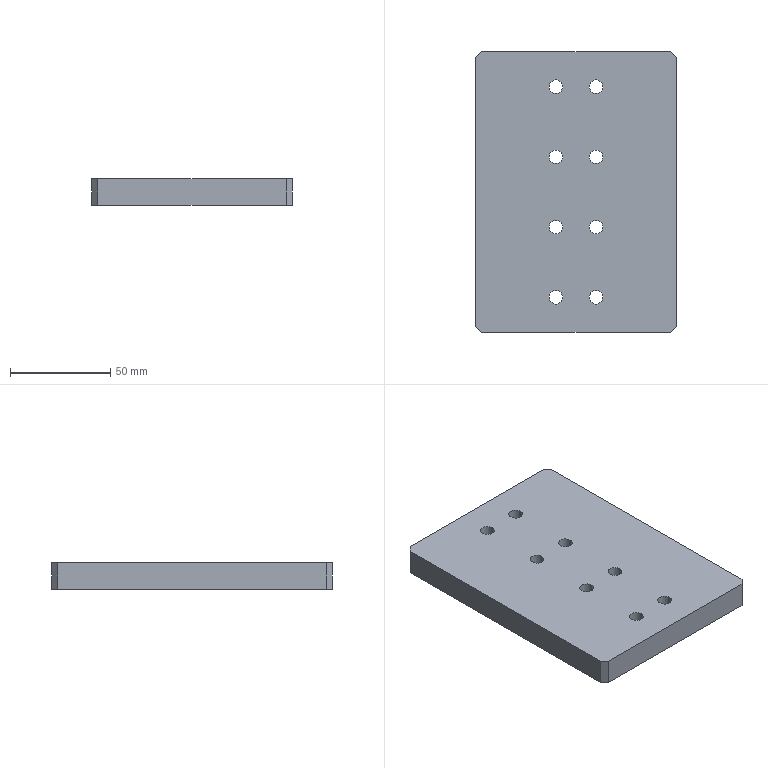Component | SolidWorks | STE21014.01-43-1 | 1 solid | 26 faces | box 100 x 140 x 13 mm | volume 177989 mm3 | cylinder 16 | plane 10 | commonest cylinder face diameters 6.8 x16 | material Q235
build123d program:
from build123d import *

# Parameters (mm, degrees)
SKETCH1_W           = 140
SKETCH1_H           = 100
BOSS_EXTRUDE1_DEPTH = 13
M8_TAPPED_HOLE1_D   = 6.8
CHAMFER1_SIZE       = 3


with BuildPart() as part:
    # Sketch1 → Boss-Extrude1 (new body)
    with BuildSketch(Plane(origin=(0, 0, 0), x_dir=(1, 0, 0), z_dir=(0, 1, 0))):
        Rectangle(SKETCH1_W, SKETCH1_H)
    extrude(amount=BOSS_EXTRUDE1_DEPTH)

    # M8 Tapped Hole1 (through all)
    with Locations(Plane(origin=(0, 13, 0), x_dir=(1, 0, 0), z_dir=(0, 1, 0))):
        with Locations((-52.5, -10), (-17.5, -10), (17.5, -10), (52.5, -10), (52.5, 10), (17.5, 10), (-17.5, 10), (-52.5, 10)):
            Hole(M8_TAPPED_HOLE1_D / 2)

    # Chamfer1
    chamfer1_edges = [part.edges().sort_by_distance(p)[0] for p in [
        (-70, 6.5, -50),
        (70, 6.5, -50),
        (70, 6.5, 50),
        (-70, 6.5, 50),
    ]]
    chamfer(chamfer1_edges, length=CHAMFER1_SIZE)


solid = part.part

# Placed as in the assembly
solid = solid.moved(Location((355, 550, -623), (90, -90, 0)))
STEP:
#1=COLOUR_RGB('',0.7922,0.8196,0.9333);
#2=FILL_AREA_STYLE_COLOUR('',#1);
#3=FILL_AREA_STYLE('',(#2));
#4=SURFACE_STYLE_FILL_AREA(#3);
#5=SURFACE_SIDE_STYLE('',(#4));
#6=SURFACE_STYLE_USAGE(.BOTH.,#5);
#7=PRESENTATION_STYLE_ASSIGNMENT((#6));
#8=CARTESIAN_POINT('',(13.717,19.587,-24.016));
#9=VERTEX_POINT('',#8);
#10=CARTESIAN_POINT('',(13.449,19.587,-24.016));
#11=VERTEX_POINT('',#10);
#12=CARTESIAN_POINT('',(13.583,19.587,-24.016));
#13=DIRECTION('',(0.,-0.,-1.));
#14=DIRECTION('',(-1.,0.,0.));
#15=AXIS2_PLACEMENT_3D('',#12,#13,#14);
#16=CIRCLE('',#15,0.1339);
#17=EDGE_CURVE('',#9,#11,#16,.T.);
#18=ORIENTED_EDGE('',*,*,#17,.F.);
#19=CARTESIAN_POINT('',(13.717,19.587,-24.528));
#20=VERTEX_POINT('',#19);
#21=CARTESIAN_POINT('',(13.717,19.587,-24.528));
#22=DIRECTION('',(0.,-0.,-1.));
#23=VECTOR('',#22,39.37);
#24=LINE('',#21,#23);
#25=EDGE_CURVE('',#9,#20,#24,.T.);
#26=ORIENTED_EDGE('',*,*,#25,.T.);
#27=CARTESIAN_POINT('',(13.449,19.587,-24.528));
#28=VERTEX_POINT('',#27);
#29=CARTESIAN_POINT('',(13.583,19.587,-24.528));
#30=DIRECTION('',(0.,-0.,-1.));
#31=DIRECTION('',(-1.,0.,0.));
#32=AXIS2_PLACEMENT_3D('',#29,#30,#31);
#33=CIRCLE('',#32,0.1339);
#34=EDGE_CURVE('',#20,#28,#33,.T.);
#35=ORIENTED_EDGE('',*,*,#34,.T.);
#36=CARTESIAN_POINT('',(13.449,19.587,-24.528));
#37=DIRECTION('',(0.,-0.,-1.));
#38=VECTOR('',#37,39.37);
#39=LINE('',#36,#38);
#40=EDGE_CURVE('',#11,#28,#39,.T.);
#41=ORIENTED_EDGE('',*,*,#40,.F.);
#42=EDGE_LOOP('',(#18,#26,#35,#41));
#43=FACE_OUTER_BOUND('',#42,.T.);
#44=CARTESIAN_POINT('',(13.583,19.587,-24.528));
#45=DIRECTION('',(0.,-0.,-1.));
#46=DIRECTION('',(-1.,0.,0.));
#47=AXIS2_PLACEMENT_3D('',#44,#45,#46);
#48=CYLINDRICAL_SURFACE('',#47,0.1339);
#49=ADVANCED_FACE('',(#43),#48,.F.);
#50=CARTESIAN_POINT('',(13.717,20.965,-24.016));
#51=VERTEX_POINT('',#50);
#52=CARTESIAN_POINT('',(13.449,20.965,-24.016));
#53=VERTEX_POINT('',#52);
#54=CARTESIAN_POINT('',(13.583,20.965,-24.016));
#55=DIRECTION('',(0.,-0.,-1.));
#56=DIRECTION('',(-1.,0.,0.));
#57=AXIS2_PLACEMENT_3D('',#54,#55,#56);
#58=CIRCLE('',#57,0.1339);
#59=EDGE_CURVE('',#51,#53,#58,.T.);
#60=ORIENTED_EDGE('',*,*,#59,.F.);
#61=CARTESIAN_POINT('',(13.717,20.965,-24.528));
#62=VERTEX_POINT('',#61);
#63=CARTESIAN_POINT('',(13.717,20.965,-24.528));
#64=DIRECTION('',(0.,-0.,-1.));
#65=VECTOR('',#64,39.37);
#66=LINE('',#63,#65);
#67=EDGE_CURVE('',#51,#62,#66,.T.);
#68=ORIENTED_EDGE('',*,*,#67,.T.);
#69=CARTESIAN_POINT('',(13.449,20.965,-24.528));
#70=VERTEX_POINT('',#69);
#71=CARTESIAN_POINT('',(13.583,20.965,-24.528));
#72=DIRECTION('',(0.,-0.,-1.));
#73=DIRECTION('',(-1.,0.,0.));
#74=AXIS2_PLACEMENT_3D('',#71,#72,#73);
#75=CIRCLE('',#74,0.1339);
#76=EDGE_CURVE('',#62,#70,#75,.T.);
#77=ORIENTED_EDGE('',*,*,#76,.T.);
#78=CARTESIAN_POINT('',(13.449,20.965,-24.528));
#79=DIRECTION('',(0.,-0.,-1.));
#80=VECTOR('',#79,39.37);
#81=LINE('',#78,#80);
#82=EDGE_CURVE('',#53,#70,#81,.T.);
#83=ORIENTED_EDGE('',*,*,#82,.F.);
#84=EDGE_LOOP('',(#60,#68,#77,#83));
#85=FACE_OUTER_BOUND('',#84,.T.);
#86=CARTESIAN_POINT('',(13.583,20.965,-24.528));
#87=DIRECTION('',(0.,-0.,-1.));
#88=DIRECTION('',(-1.,0.,0.));
#89=AXIS2_PLACEMENT_3D('',#86,#87,#88);
#90=CYLINDRICAL_SURFACE('',#89,0.1339);
#91=ADVANCED_FACE('',(#85),#90,.F.);
#92=CARTESIAN_POINT('',(13.717,22.343,-24.016));
#93=VERTEX_POINT('',#92);
#94=CARTESIAN_POINT('',(13.449,22.343,-24.016));
#95=VERTEX_POINT('',#94);
#96=CARTESIAN_POINT('',(13.583,22.343,-24.016));
#97=DIRECTION('',(0.,-0.,-1.));
#98=DIRECTION('',(-1.,0.,0.));
#99=AXIS2_PLACEMENT_3D('',#96,#97,#98);
#100=CIRCLE('',#99,0.1339);
#101=EDGE_CURVE('',#93,#95,#100,.T.);
#102=ORIENTED_EDGE('',*,*,#101,.F.);
#103=CARTESIAN_POINT('',(13.717,22.343,-24.528));
#104=VERTEX_POINT('',#103);
#105=CARTESIAN_POINT('',(13.717,22.343,-24.528));
#106=DIRECTION('',(0.,-0.,-1.));
#107=VECTOR('',#106,39.37);
#108=LINE('',#105,#107);
#109=EDGE_CURVE('',#93,#104,#108,.T.);
#110=ORIENTED_EDGE('',*,*,#109,.T.);
#111=CARTESIAN_POINT('',(13.449,22.343,-24.528));
#112=VERTEX_POINT('',#111);
#113=CARTESIAN_POINT('',(13.583,22.343,-24.528));
#114=DIRECTION('',(0.,-0.,-1.));
#115=DIRECTION('',(-1.,0.,0.));
#116=AXIS2_PLACEMENT_3D('',#113,#114,#115);
#117=CIRCLE('',#116,0.1339);
#118=EDGE_CURVE('',#104,#112,#117,.T.);
#119=ORIENTED_EDGE('',*,*,#118,.T.);
#120=CARTESIAN_POINT('',(13.449,22.343,-24.528));
#121=DIRECTION('',(0.,-0.,-1.));
#122=VECTOR('',#121,39.37);
#123=LINE('',#120,#122);
#124=EDGE_CURVE('',#95,#112,#123,.T.);
#125=ORIENTED_EDGE('',*,*,#124,.F.);
#126=EDGE_LOOP('',(#102,#110,#119,#125));
#127=FACE_OUTER_BOUND('',#126,.T.);
#128=CARTESIAN_POINT('',(13.583,22.343,-24.528));
#129=DIRECTION('',(0.,-0.,-1.));
#130=DIRECTION('',(-1.,0.,0.));
#131=AXIS2_PLACEMENT_3D('',#128,#129,#130);
#132=CYLINDRICAL_SURFACE('',#131,0.1339);
#133=ADVANCED_FACE('',(#127),#132,.F.);
#134=CARTESIAN_POINT('',(13.717,23.72,-24.016));
#135=VERTEX_POINT('',#134);
#136=CARTESIAN_POINT('',(13.449,23.72,-24.016));
#137=VERTEX_POINT('',#136);
#138=CARTESIAN_POINT('',(13.583,23.72,-24.016));
#139=DIRECTION('',(0.,-0.,-1.));
#140=DIRECTION('',(-1.,0.,0.));
#141=AXIS2_PLACEMENT_3D('',#138,#139,#140);
#142=CIRCLE('',#141,0.1339);
#143=EDGE_CURVE('',#135,#137,#142,.T.);
#144=ORIENTED_EDGE('',*,*,#143,.F.);
#145=CARTESIAN_POINT('',(13.717,23.72,-24.528));
#146=VERTEX_POINT('',#145);
#147=CARTESIAN_POINT('',(13.717,23.72,-24.528));
#148=DIRECTION('',(0.,-0.,-1.));
#149=VECTOR('',#148,39.37);
#150=LINE('',#147,#149);
#151=EDGE_CURVE('',#135,#146,#150,.T.);
#152=ORIENTED_EDGE('',*,*,#151,.T.);
#153=CARTESIAN_POINT('',(13.449,23.72,-24.528));
#154=VERTEX_POINT('',#153);
#155=CARTESIAN_POINT('',(13.583,23.72,-24.528));
#156=DIRECTION('',(0.,-0.,-1.));
#157=DIRECTION('',(-1.,0.,0.));
#158=AXIS2_PLACEMENT_3D('',#155,#156,#157);
#159=CIRCLE('',#158,0.1339);
#160=EDGE_CURVE('',#146,#154,#159,.T.);
#161=ORIENTED_EDGE('',*,*,#160,.T.);
#162=CARTESIAN_POINT('',(13.449,23.72,-24.528));
#163=DIRECTION('',(0.,-0.,-1.));
#164=VECTOR('',#163,39.37);
#165=LINE('',#162,#164);
#166=EDGE_CURVE('',#137,#154,#165,.T.);
#167=ORIENTED_EDGE('',*,*,#166,.F.);
#168=EDGE_LOOP('',(#144,#152,#161,#167));
#169=FACE_OUTER_BOUND('',#168,.T.);
#170=CARTESIAN_POINT('',(13.583,23.72,-24.528));
#171=DIRECTION('',(0.,-0.,-1.));
#172=DIRECTION('',(-1.,0.,0.));
#173=AXIS2_PLACEMENT_3D('',#170,#171,#172);
#174=CYLINDRICAL_SURFACE('',#173,0.1339);
#175=ADVANCED_FACE('',(#169),#174,.F.);
#176=CARTESIAN_POINT('',(14.504,23.72,-24.016));
#177=VERTEX_POINT('',#176);
#178=CARTESIAN_POINT('',(14.236,23.72,-24.016));
#179=VERTEX_POINT('',#178);
#180=CARTESIAN_POINT('',(14.37,23.72,-24.016));
#181=DIRECTION('',(0.,-0.,-1.));
#182=DIRECTION('',(-1.,0.,0.));
#183=AXIS2_PLACEMENT_3D('',#180,#181,#182);
#184=CIRCLE('',#183,0.1339);
#185=EDGE_CURVE('',#177,#179,#184,.T.);
#186=ORIENTED_EDGE('',*,*,#185,.F.);
#187=CARTESIAN_POINT('',(14.504,23.72,-24.528));
#188=VERTEX_POINT('',#187);
#189=CARTESIAN_POINT('',(14.504,23.72,-24.528));
#190=DIRECTION('',(0.,-0.,-1.));
#191=VECTOR('',#190,39.37);
#192=LINE('',#189,#191);
#193=EDGE_CURVE('',#177,#188,#192,.T.);
#194=ORIENTED_EDGE('',*,*,#193,.T.);
#195=CARTESIAN_POINT('',(14.236,23.72,-24.528));
#196=VERTEX_POINT('',#195);
#197=CARTESIAN_POINT('',(14.37,23.72,-24.528));
#198=DIRECTION('',(0.,-0.,-1.));
#199=DIRECTION('',(-1.,0.,0.));
#200=AXIS2_PLACEMENT_3D('',#197,#198,#199);
#201=CIRCLE('',#200,0.1339);
#202=EDGE_CURVE('',#188,#196,#201,.T.);
#203=ORIENTED_EDGE('',*,*,#202,.T.);
#204=CARTESIAN_POINT('',(14.236,23.72,-24.528));
#205=DIRECTION('',(0.,-0.,-1.));
#206=VECTOR('',#205,39.37);
#207=LINE('',#204,#206);
#208=EDGE_CURVE('',#179,#196,#207,.T.);
#209=ORIENTED_EDGE('',*,*,#208,.F.);
#210=EDGE_LOOP('',(#186,#194,#203,#209));
#211=FACE_OUTER_BOUND('',#210,.T.);
#212=CARTESIAN_POINT('',(14.37,23.72,-24.528));
#213=DIRECTION('',(0.,-0.,-1.));
#214=DIRECTION('',(-1.,0.,0.));
#215=AXIS2_PLACEMENT_3D('',#212,#213,#214);
#216=CYLINDRICAL_SURFACE('',#215,0.1339);
#217=ADVANCED_FACE('',(#211),#216,.F.);
#218=CARTESIAN_POINT('',(14.504,22.343,-24.016));
#219=VERTEX_POINT('',#218);
#220=CARTESIAN_POINT('',(14.236,22.343,-24.016));
#221=VERTEX_POINT('',#220);
#222=CARTESIAN_POINT('',(14.37,22.343,-24.016));
#223=DIRECTION('',(0.,-0.,-1.));
#224=DIRECTION('',(-1.,0.,0.));
#225=AXIS2_PLACEMENT_3D('',#222,#223,#224);
#226=CIRCLE('',#225,0.1339);
#227=EDGE_CURVE('',#219,#221,#226,.T.);
#228=ORIENTED_EDGE('',*,*,#227,.F.);
#229=CARTESIAN_POINT('',(14.504,22.343,-24.528));
#230=VERTEX_POINT('',#229);
#231=CARTESIAN_POINT('',(14.504,22.343,-24.528));
#232=DIRECTION('',(0.,-0.,-1.));
#233=VECTOR('',#232,39.37);
#234=LINE('',#231,#233);
#235=EDGE_CURVE('',#219,#230,#234,.T.);
#236=ORIENTED_EDGE('',*,*,#235,.T.);
#237=CARTESIAN_POINT('',(14.236,22.343,-24.528));
#238=VERTEX_POINT('',#237);
#239=CARTESIAN_POINT('',(14.37,22.343,-24.528));
#240=DIRECTION('',(0.,-0.,-1.));
#241=DIRECTION('',(-1.,0.,0.));
#242=AXIS2_PLACEMENT_3D('',#239,#240,#241);
#243=CIRCLE('',#242,0.1339);
#244=EDGE_CURVE('',#230,#238,#243,.T.);
#245=ORIENTED_EDGE('',*,*,#244,.T.);
#246=CARTESIAN_POINT('',(14.236,22.343,-24.528));
#247=DIRECTION('',(0.,-0.,-1.));
#248=VECTOR('',#247,39.37);
#249=LINE('',#246,#248);
#250=EDGE_CURVE('',#221,#238,#249,.T.);
#251=ORIENTED_EDGE('',*,*,#250,.F.);
#252=EDGE_LOOP('',(#228,#236,#245,#251));
#253=FACE_OUTER_BOUND('',#252,.T.);
#254=CARTESIAN_POINT('',(14.37,22.343,-24.528));
#255=DIRECTION('',(0.,-0.,-1.));
#256=DIRECTION('',(-1.,0.,0.));
#257=AXIS2_PLACEMENT_3D('',#254,#255,#256);
#258=CYLINDRICAL_SURFACE('',#257,0.1339);
#259=ADVANCED_FACE('',(#253),#258,.F.);
#260=CARTESIAN_POINT('',(14.504,20.965,-24.016));
#261=VERTEX_POINT('',#260);
#262=CARTESIAN_POINT('',(14.236,20.965,-24.016));
#263=VERTEX_POINT('',#262);
#264=CARTESIAN_POINT('',(14.37,20.965,-24.016));
#265=DIRECTION('',(0.,-0.,-1.));
#266=DIRECTION('',(-1.,0.,0.));
#267=AXIS2_PLACEMENT_3D('',#264,#265,#266);
#268=CIRCLE('',#267,0.1339);
#269=EDGE_CURVE('',#261,#263,#268,.T.);
#270=ORIENTED_EDGE('',*,*,#269,.F.);
#271=CARTESIAN_POINT('',(14.504,20.965,-24.528));
#272=VERTEX_POINT('',#271);
#273=CARTESIAN_POINT('',(14.504,20.965,-24.528));
#274=DIRECTION('',(0.,-0.,-1.));
#275=VECTOR('',#274,39.37);
#276=LINE('',#273,#275);
#277=EDGE_CURVE('',#261,#272,#276,.T.);
#278=ORIENTED_EDGE('',*,*,#277,.T.);
#279=CARTESIAN_POINT('',(14.236,20.965,-24.528));
#280=VERTEX_POINT('',#279);
#281=CARTESIAN_POINT('',(14.37,20.965,-24.528));
#282=DIRECTION('',(0.,-0.,-1.));
#283=DIRECTION('',(-1.,0.,0.));
#284=AXIS2_PLACEMENT_3D('',#281,#282,#283);
#285=CIRCLE('',#284,0.1339);
#286=EDGE_CURVE('',#272,#280,#285,.T.);
#287=ORIENTED_EDGE('',*,*,#286,.T.);
#288=CARTESIAN_POINT('',(14.236,20.965,-24.528));
#289=DIRECTION('',(0.,-0.,-1.));
#290=VECTOR('',#289,39.37);
#291=LINE('',#288,#290);
#292=EDGE_CURVE('',#263,#280,#291,.T.);
#293=ORIENTED_EDGE('',*,*,#292,.F.);
#294=EDGE_LOOP('',(#270,#278,#287,#293));
#295=FACE_OUTER_BOUND('',#294,.T.);
#296=CARTESIAN_POINT('',(14.37,20.965,-24.528));
#297=DIRECTION('',(0.,-0.,-1.));
#298=DIRECTION('',(-1.,0.,0.));
#299=AXIS2_PLACEMENT_3D('',#296,#297,#298);
#300=CYLINDRICAL_SURFACE('',#299,0.1339);
#301=ADVANCED_FACE('',(#295),#300,.F.);
#302=CARTESIAN_POINT('',(14.504,19.587,-24.016));
#303=VERTEX_POINT('',#302);
#304=CARTESIAN_POINT('',(14.236,19.587,-24.016));
#305=VERTEX_POINT('',#304);
#306=CARTESIAN_POINT('',(14.37,19.587,-24.016));
#307=DIRECTION('',(0.,-0.,-1.));
#308=DIRECTION('',(-1.,0.,0.));
#309=AXIS2_PLACEMENT_3D('',#306,#307,#308);
#310=CIRCLE('',#309,0.1339);
#311=EDGE_CURVE('',#303,#305,#310,.T.);
#312=ORIENTED_EDGE('',*,*,#311,.F.);
#313=CARTESIAN_POINT('',(14.504,19.587,-24.528));
#314=VERTEX_POINT('',#313);
#315=CARTESIAN_POINT('',(14.504,19.587,-24.528));
#316=DIRECTION('',(0.,-0.,-1.));
#317=VECTOR('',#316,39.37);
#318=LINE('',#315,#317);
#319=EDGE_CURVE('',#303,#314,#318,.T.);
#320=ORIENTED_EDGE('',*,*,#319,.T.);
#321=CARTESIAN_POINT('',(14.236,19.587,-24.528));
#322=VERTEX_POINT('',#321);
#323=CARTESIAN_POINT('',(14.37,19.587,-24.528));
#324=DIRECTION('',(0.,-0.,-1.));
#325=DIRECTION('',(-1.,0.,0.));
#326=AXIS2_PLACEMENT_3D('',#323,#324,#325);
#327=CIRCLE('',#326,0.1339);
#328=EDGE_CURVE('',#314,#322,#327,.T.);
#329=ORIENTED_EDGE('',*,*,#328,.T.);
#330=CARTESIAN_POINT('',(14.236,19.587,-24.528));
#331=DIRECTION('',(0.,-0.,-1.));
#332=VECTOR('',#331,39.37);
#333=LINE('',#330,#332);
#334=EDGE_CURVE('',#305,#322,#333,.T.);
#335=ORIENTED_EDGE('',*,*,#334,.F.);
#336=EDGE_LOOP('',(#312,#320,#329,#335));
#337=FACE_OUTER_BOUND('',#336,.T.);
#338=CARTESIAN_POINT('',(14.37,19.587,-24.528));
#339=DIRECTION('',(0.,-0.,-1.));
#340=DIRECTION('',(-1.,0.,0.));
#341=AXIS2_PLACEMENT_3D('',#338,#339,#340);
#342=CYLINDRICAL_SURFACE('',#341,0.1339);
#343=ADVANCED_FACE('',(#337),#342,.F.);
#344=CARTESIAN_POINT('',(15.827,18.898,-24.528));
#345=VERTEX_POINT('',#344);
#346=CARTESIAN_POINT('',(12.126,18.898,-24.528));
#347=VERTEX_POINT('',#346);
#348=CARTESIAN_POINT('',(12.008,18.898,-24.528));
#349=DIRECTION('',(-1.,0.,-0.));
#350=VECTOR('',#349,39.37);
#351=LINE('',#348,#350);
#352=EDGE_CURVE('',#345,#347,#351,.T.);
#353=ORIENTED_EDGE('',*,*,#352,.F.);
#354=CARTESIAN_POINT('',(15.827,18.898,-24.016));
#355=VERTEX_POINT('',#354);
#356=CARTESIAN_POINT('',(15.827,18.898,-24.528));
#357=DIRECTION('',(-0.,0.,1.));
#358=VECTOR('',#357,39.37);
#359=LINE('',#356,#358);
#360=EDGE_CURVE('',#345,#355,#359,.T.);
#361=ORIENTED_EDGE('',*,*,#360,.T.);
#362=CARTESIAN_POINT('',(12.126,18.898,-24.016));
#363=VERTEX_POINT('',#362);
#364=CARTESIAN_POINT('',(12.008,18.898,-24.016));
#365=DIRECTION('',(-1.,0.,-0.));
#366=VECTOR('',#365,39.37);
#367=LINE('',#364,#366);
#368=EDGE_CURVE('',#355,#363,#367,.T.);
#369=ORIENTED_EDGE('',*,*,#368,.T.);
#370=CARTESIAN_POINT('',(12.126,18.898,-24.528));
#371=DIRECTION('',(0.,-0.,-1.));
#372=VECTOR('',#371,39.37);
#373=LINE('',#370,#372);
#374=EDGE_CURVE('',#363,#347,#373,.T.);
#375=ORIENTED_EDGE('',*,*,#374,.T.);
#376=EDGE_LOOP('',(#353,#361,#369,#375));
#377=FACE_OUTER_BOUND('',#376,.T.);
#378=CARTESIAN_POINT('',(12.008,18.898,-24.528));
#379=DIRECTION('',(0.,1.,-0.));
#380=DIRECTION('',(1.,-0.,0.));
#381=AXIS2_PLACEMENT_3D('',#378,#379,#380);
#382=PLANE('',#381);
#383=ADVANCED_FACE('',(#377),#382,.F.);
#384=CARTESIAN_POINT('',(12.008,19.016,-24.016));
#385=VERTEX_POINT('',#384);
#386=CARTESIAN_POINT('',(12.008,24.291,-24.016));
#387=VERTEX_POINT('',#386);
#388=CARTESIAN_POINT('',(12.008,24.409,-24.016));
#389=DIRECTION('',(0.,1.,-0.));
#390=VECTOR('',#389,39.37);
#391=LINE('',#388,#390);
#392=EDGE_CURVE('',#385,#387,#391,.T.);
#393=ORIENTED_EDGE('',*,*,#392,.T.);
#394=CARTESIAN_POINT('',(12.008,24.291,-24.528));
#395=VERTEX_POINT('',#394);
#396=CARTESIAN_POINT('',(12.008,24.291,-24.528));
#397=DIRECTION('',(0.,-0.,-1.));
#398=VECTOR('',#397,39.37);
#399=LINE('',#396,#398);
#400=EDGE_CURVE('',#387,#395,#399,.T.);
#401=ORIENTED_EDGE('',*,*,#400,.T.);
#402=CARTESIAN_POINT('',(12.008,19.016,-24.528));
#403=VERTEX_POINT('',#402);
#404=CARTESIAN_POINT('',(12.008,24.409,-24.528));
#405=DIRECTION('',(0.,1.,-0.));
#406=VECTOR('',#405,39.37);
#407=LINE('',#404,#406);
#408=EDGE_CURVE('',#403,#395,#407,.T.);
#409=ORIENTED_EDGE('',*,*,#408,.F.);
#410=CARTESIAN_POINT('',(12.008,19.016,-24.528));
#411=DIRECTION('',(-0.,0.,1.));
#412=VECTOR('',#411,39.37);
#413=LINE('',#410,#412);
#414=EDGE_CURVE('',#403,#385,#413,.T.);
#415=ORIENTED_EDGE('',*,*,#414,.T.);
#416=EDGE_LOOP('',(#393,#401,#409,#415));
#417=FACE_OUTER_BOUND('',#416,.T.);
#418=CARTESIAN_POINT('',(12.008,24.409,-24.528));
#419=DIRECTION('',(1.,-0.,0.));
#420=DIRECTION('',(-0.,-1.,0.));
#421=AXIS2_PLACEMENT_3D('',#418,#419,#420);
#422=PLANE('',#421);
#423=ADVANCED_FACE('',(#417),#422,.F.);
#424=CARTESIAN_POINT('',(12.126,24.409,-24.528));
#425=VERTEX_POINT('',#424);
#426=CARTESIAN_POINT('',(15.827,24.409,-24.528));
#427=VERTEX_POINT('',#426);
#428=CARTESIAN_POINT('',(12.008,24.409,-24.528));
#429=DIRECTION('',(1.,-0.,0.));
#430=VECTOR('',#429,39.37);
#431=LINE('',#428,#430);
#432=EDGE_CURVE('',#425,#427,#431,.T.);
#433=ORIENTED_EDGE('',*,*,#432,.F.);
#434=CARTESIAN_POINT('',(12.126,24.409,-24.016));
#435=VERTEX_POINT('',#434);
#436=CARTESIAN_POINT('',(12.126,24.409,-24.528));
#437=DIRECTION('',(-0.,0.,1.));
#438=VECTOR('',#437,39.37);
#439=LINE('',#436,#438);
#440=EDGE_CURVE('',#425,#435,#439,.T.);
#441=ORIENTED_EDGE('',*,*,#440,.T.);
#442=CARTESIAN_POINT('',(15.827,24.409,-24.016));
#443=VERTEX_POINT('',#442);
#444=CARTESIAN_POINT('',(12.008,24.409,-24.016));
#445=DIRECTION('',(1.,-0.,0.));
#446=VECTOR('',#445,39.37);
#447=LINE('',#444,#446);
#448=EDGE_CURVE('',#435,#443,#447,.T.);
#449=ORIENTED_EDGE('',*,*,#448,.T.);
#450=CARTESIAN_POINT('',(15.827,24.409,-24.528));
#451=DIRECTION('',(0.,-0.,-1.));
#452=VECTOR('',#451,39.37);
#453=LINE('',#450,#452);
#454=EDGE_CURVE('',#443,#427,#453,.T.);
#455=ORIENTED_EDGE('',*,*,#454,.T.);
#456=EDGE_LOOP('',(#433,#441,#449,#455));
#457=FACE_OUTER_BOUND('',#456,.T.);
#458=CARTESIAN_POINT('',(12.008,24.409,-24.528));
#459=DIRECTION('',(-0.,-1.,0.));
#460=DIRECTION('',(-1.,0.,-0.));
#461=AXIS2_PLACEMENT_3D('',#458,#459,#460);
#462=PLANE('',#461);
#463=ADVANCED_FACE('',(#457),#462,.F.);
#464=CARTESIAN_POINT('',(15.945,24.291,-24.528));
#465=VERTEX_POINT('',#464);
#466=CARTESIAN_POINT('',(15.945,19.016,-24.528));
#467=VERTEX_POINT('',#466);
#468=CARTESIAN_POINT('',(15.945,24.409,-24.528));
#469=DIRECTION('',(-0.,-1.,0.));
#470=VECTOR('',#469,39.37);
#471=LINE('',#468,#470);
#472=EDGE_CURVE('',#465,#467,#471,.T.);
#473=ORIENTED_EDGE('',*,*,#472,.F.);
#474=CARTESIAN_POINT('',(15.945,24.291,-24.016));
#475=VERTEX_POINT('',#474);
#476=CARTESIAN_POINT('',(15.945,24.291,-24.528));
#477=DIRECTION('',(-0.,0.,1.));
#478=VECTOR('',#477,39.37);
#479=LINE('',#476,#478);
#480=EDGE_CURVE('',#465,#475,#479,.T.);
#481=ORIENTED_EDGE('',*,*,#480,.T.);
#482=CARTESIAN_POINT('',(15.945,19.016,-24.016));
#483=VERTEX_POINT('',#482);
#484=CARTESIAN_POINT('',(15.945,24.409,-24.016));
#485=DIRECTION('',(-0.,-1.,0.));
#486=VECTOR('',#485,39.37);
#487=LINE('',#484,#486);
#488=EDGE_CURVE('',#475,#483,#487,.T.);
#489=ORIENTED_EDGE('',*,*,#488,.T.);
#490=CARTESIAN_POINT('',(15.945,19.016,-24.528));
#491=DIRECTION('',(0.,-0.,-1.));
#492=VECTOR('',#491,39.37);
#493=LINE('',#490,#492);
#494=EDGE_CURVE('',#483,#467,#493,.T.);
#495=ORIENTED_EDGE('',*,*,#494,.T.);
#496=EDGE_LOOP('',(#473,#481,#489,#495));
#497=FACE_OUTER_BOUND('',#496,.T.);
#498=CARTESIAN_POINT('',(15.945,24.409,-24.528));
#499=DIRECTION('',(-1.,0.,-0.));
#500=DIRECTION('',(0.,1.,-0.));
#501=AXIS2_PLACEMENT_3D('',#498,#499,#500);
#502=PLANE('',#501);
#503=ADVANCED_FACE('',(#497),#502,.F.);
#504=CARTESIAN_POINT('',(13.583,19.587,-24.528));
#505=DIRECTION('',(0.,-0.,-1.));
#506=DIRECTION('',(-1.,0.,0.));
#507=AXIS2_PLACEMENT_3D('',#504,#505,#506);
#508=CIRCLE('',#507,0.1339);
#509=EDGE_CURVE('',#28,#20,#508,.T.);
#510=ORIENTED_EDGE('',*,*,#509,.F.);
#511=ORIENTED_EDGE('',*,*,#34,.F.);
#512=EDGE_LOOP('',(#510,#511));
#513=FACE_BOUND('',#512,.T.);
#514=CARTESIAN_POINT('',(13.583,20.965,-24.528));
#515=DIRECTION('',(0.,-0.,-1.));
#516=DIRECTION('',(-1.,0.,0.));
#517=AXIS2_PLACEMENT_3D('',#514,#515,#516);
#518=CIRCLE('',#517,0.1339);
#519=EDGE_CURVE('',#70,#62,#518,.T.);
#520=ORIENTED_EDGE('',*,*,#519,.F.);
#521=ORIENTED_EDGE('',*,*,#76,.F.);
#522=EDGE_LOOP('',(#520,#521));
#523=FACE_BOUND('',#522,.T.);
#524=CARTESIAN_POINT('',(13.583,22.343,-24.528));
#525=DIRECTION('',(0.,-0.,-1.));
#526=DIRECTION('',(-1.,0.,0.));
#527=AXIS2_PLACEMENT_3D('',#524,#525,#526);
#528=CIRCLE('',#527,0.1339);
#529=EDGE_CURVE('',#112,#104,#528,.T.);
#530=ORIENTED_EDGE('',*,*,#529,.F.);
#531=ORIENTED_EDGE('',*,*,#118,.F.);
#532=EDGE_LOOP('',(#530,#531));
#533=FACE_BOUND('',#532,.T.);
#534=CARTESIAN_POINT('',(13.583,23.72,-24.528));
#535=DIRECTION('',(0.,-0.,-1.));
#536=DIRECTION('',(-1.,0.,0.));
#537=AXIS2_PLACEMENT_3D('',#534,#535,#536);
#538=CIRCLE('',#537,0.1339);
#539=EDGE_CURVE('',#154,#146,#538,.T.);
#540=ORIENTED_EDGE('',*,*,#539,.F.);
#541=ORIENTED_EDGE('',*,*,#160,.F.);
#542=EDGE_LOOP('',(#540,#541));
#543=FACE_BOUND('',#542,.T.);
#544=CARTESIAN_POINT('',(14.37,23.72,-24.528));
#545=DIRECTION('',(0.,-0.,-1.));
#546=DIRECTION('',(-1.,0.,0.));
#547=AXIS2_PLACEMENT_3D('',#544,#545,#546);
#548=CIRCLE('',#547,0.1339);
#549=EDGE_CURVE('',#196,#188,#548,.T.);
#550=ORIENTED_EDGE('',*,*,#549,.F.);
#551=ORIENTED_EDGE('',*,*,#202,.F.);
#552=EDGE_LOOP('',(#550,#551));
#553=FACE_BOUND('',#552,.T.);
#554=CARTESIAN_POINT('',(14.37,22.343,-24.528));
#555=DIRECTION('',(0.,-0.,-1.));
#556=DIRECTION('',(-1.,0.,0.));
#557=AXIS2_PLACEMENT_3D('',#554,#555,#556);
#558=CIRCLE('',#557,0.1339);
#559=EDGE_CURVE('',#238,#230,#558,.T.);
#560=ORIENTED_EDGE('',*,*,#559,.F.);
#561=ORIENTED_EDGE('',*,*,#244,.F.);
#562=EDGE_LOOP('',(#560,#561));
#563=FACE_BOUND('',#562,.T.);
#564=CARTESIAN_POINT('',(14.37,20.965,-24.528));
#565=DIRECTION('',(0.,-0.,-1.));
#566=DIRECTION('',(-1.,0.,0.));
#567=AXIS2_PLACEMENT_3D('',#564,#565,#566);
#568=CIRCLE('',#567,0.1339);
#569=EDGE_CURVE('',#280,#272,#568,.T.);
#570=ORIENTED_EDGE('',*,*,#569,.F.);
#571=ORIENTED_EDGE('',*,*,#286,.F.);
#572=EDGE_LOOP('',(#570,#571));
#573=FACE_BOUND('',#572,.T.);
#574=CARTESIAN_POINT('',(14.37,19.587,-24.528));
#575=DIRECTION('',(0.,-0.,-1.));
#576=DIRECTION('',(-1.,0.,0.));
#577=AXIS2_PLACEMENT_3D('',#574,#575,#576);
#578=CIRCLE('',#577,0.1339);
#579=EDGE_CURVE('',#322,#314,#578,.T.);
#580=ORIENTED_EDGE('',*,*,#579,.F.);
#581=ORIENTED_EDGE('',*,*,#328,.F.);
#582=EDGE_LOOP('',(#580,#581));
#583=FACE_BOUND('',#582,.T.);
#584=ORIENTED_EDGE('',*,*,#408,.T.);
#585=CARTESIAN_POINT('',(11.673,23.957,-24.528));
#586=DIRECTION('',(0.7071,0.7071,-0.));
#587=VECTOR('',#586,39.37);
#588=LINE('',#585,#587);
#589=EDGE_CURVE('',#395,#425,#588,.T.);
#590=ORIENTED_EDGE('',*,*,#589,.T.);
#591=ORIENTED_EDGE('',*,*,#432,.T.);
#592=CARTESIAN_POINT('',(16.28,23.957,-24.528));
#593=DIRECTION('',(0.7071,-0.7071,0.));
#594=VECTOR('',#593,39.37);
#595=LINE('',#592,#594);
#596=EDGE_CURVE('',#427,#465,#595,.T.);
#597=ORIENTED_EDGE('',*,*,#596,.T.);
#598=ORIENTED_EDGE('',*,*,#472,.T.);
#599=CARTESIAN_POINT('',(16.28,19.35,-24.528));
#600=DIRECTION('',(-0.7071,-0.7071,0.));
#601=VECTOR('',#600,39.37);
#602=LINE('',#599,#601);
#603=EDGE_CURVE('',#467,#345,#602,.T.);
#604=ORIENTED_EDGE('',*,*,#603,.T.);
#605=ORIENTED_EDGE('',*,*,#352,.T.);
#606=CARTESIAN_POINT('',(11.673,19.35,-24.528));
#607=DIRECTION('',(-0.7071,0.7071,-0.));
#608=VECTOR('',#607,39.37);
#609=LINE('',#606,#608);
#610=EDGE_CURVE('',#347,#403,#609,.T.);
#611=ORIENTED_EDGE('',*,*,#610,.T.);
#612=EDGE_LOOP('',(#584,#590,#591,#597,#598,#604,#605,#611));
#613=FACE_OUTER_BOUND('',#612,.T.);
#614=CARTESIAN_POINT('',(13.976,21.654,-24.528));
#615=DIRECTION('',(0.,-0.,-1.));
#616=DIRECTION('',(-1.,0.,-0.));
#617=AXIS2_PLACEMENT_3D('',#614,#615,#616);
#618=PLANE('',#617);
#619=ADVANCED_FACE('',(#513,#523,#533,#543,#553,#563,#573,#583,#613),#618,.T.);
#620=CARTESIAN_POINT('',(13.583,19.587,-24.016));
#621=DIRECTION('',(0.,-0.,-1.));
#622=DIRECTION('',(-1.,0.,0.));
#623=AXIS2_PLACEMENT_3D('',#620,#621,#622);
#624=CIRCLE('',#623,0.1339);
#625=EDGE_CURVE('',#11,#9,#624,.T.);
#626=ORIENTED_EDGE('',*,*,#625,.T.);
#627=ORIENTED_EDGE('',*,*,#17,.T.);
#628=EDGE_LOOP('',(#626,#627));
#629=FACE_BOUND('',#628,.T.);
#630=CARTESIAN_POINT('',(13.583,20.965,-24.016));
#631=DIRECTION('',(0.,-0.,-1.));
#632=DIRECTION('',(-1.,0.,0.));
#633=AXIS2_PLACEMENT_3D('',#630,#631,#632);
#634=CIRCLE('',#633,0.1339);
#635=EDGE_CURVE('',#53,#51,#634,.T.);
#636=ORIENTED_EDGE('',*,*,#635,.T.);
#637=ORIENTED_EDGE('',*,*,#59,.T.);
#638=EDGE_LOOP('',(#636,#637));
#639=FACE_BOUND('',#638,.T.);
#640=CARTESIAN_POINT('',(13.583,22.343,-24.016));
#641=DIRECTION('',(0.,-0.,-1.));
#642=DIRECTION('',(-1.,0.,0.));
#643=AXIS2_PLACEMENT_3D('',#640,#641,#642);
#644=CIRCLE('',#643,0.1339);
#645=EDGE_CURVE('',#95,#93,#644,.T.);
#646=ORIENTED_EDGE('',*,*,#645,.T.);
#647=ORIENTED_EDGE('',*,*,#101,.T.);
#648=EDGE_LOOP('',(#646,#647));
#649=FACE_BOUND('',#648,.T.);
#650=CARTESIAN_POINT('',(13.583,23.72,-24.016));
#651=DIRECTION('',(0.,-0.,-1.));
#652=DIRECTION('',(-1.,0.,0.));
#653=AXIS2_PLACEMENT_3D('',#650,#651,#652);
#654=CIRCLE('',#653,0.1339);
#655=EDGE_CURVE('',#137,#135,#654,.T.);
#656=ORIENTED_EDGE('',*,*,#655,.T.);
#657=ORIENTED_EDGE('',*,*,#143,.T.);
#658=EDGE_LOOP('',(#656,#657));
#659=FACE_BOUND('',#658,.T.);
#660=CARTESIAN_POINT('',(14.37,23.72,-24.016));
#661=DIRECTION('',(0.,-0.,-1.));
#662=DIRECTION('',(-1.,0.,0.));
#663=AXIS2_PLACEMENT_3D('',#660,#661,#662);
#664=CIRCLE('',#663,0.1339);
#665=EDGE_CURVE('',#179,#177,#664,.T.);
#666=ORIENTED_EDGE('',*,*,#665,.T.);
#667=ORIENTED_EDGE('',*,*,#185,.T.);
#668=EDGE_LOOP('',(#666,#667));
#669=FACE_BOUND('',#668,.T.);
#670=CARTESIAN_POINT('',(14.37,22.343,-24.016));
#671=DIRECTION('',(0.,-0.,-1.));
#672=DIRECTION('',(-1.,0.,0.));
#673=AXIS2_PLACEMENT_3D('',#670,#671,#672);
#674=CIRCLE('',#673,0.1339);
#675=EDGE_CURVE('',#221,#219,#674,.T.);
#676=ORIENTED_EDGE('',*,*,#675,.T.);
#677=ORIENTED_EDGE('',*,*,#227,.T.);
#678=EDGE_LOOP('',(#676,#677));
#679=FACE_BOUND('',#678,.T.);
#680=CARTESIAN_POINT('',(14.37,20.965,-24.016));
#681=DIRECTION('',(0.,-0.,-1.));
#682=DIRECTION('',(-1.,0.,0.));
#683=AXIS2_PLACEMENT_3D('',#680,#681,#682);
#684=CIRCLE('',#683,0.1339);
#685=EDGE_CURVE('',#263,#261,#684,.T.);
#686=ORIENTED_EDGE('',*,*,#685,.T.);
#687=ORIENTED_EDGE('',*,*,#269,.T.);
#688=EDGE_LOOP('',(#686,#687));
#689=FACE_BOUND('',#688,.T.);
#690=CARTESIAN_POINT('',(14.37,19.587,-24.016));
#691=DIRECTION('',(0.,-0.,-1.));
#692=DIRECTION('',(-1.,0.,0.));
#693=AXIS2_PLACEMENT_3D('',#690,#691,#692);
#694=CIRCLE('',#693,0.1339);
#695=EDGE_CURVE('',#305,#303,#694,.T.);
#696=ORIENTED_EDGE('',*,*,#695,.T.);
#697=ORIENTED_EDGE('',*,*,#311,.T.);
#698=EDGE_LOOP('',(#696,#697));
#699=FACE_BOUND('',#698,.T.);
#700=ORIENTED_EDGE('',*,*,#448,.F.);
#701=CARTESIAN_POINT('',(12.126,24.409,-24.016));
#702=DIRECTION('',(-0.7071,-0.7071,0.));
#703=VECTOR('',#702,39.37);
#704=LINE('',#701,#703);
#705=EDGE_CURVE('',#435,#387,#704,.T.);
#706=ORIENTED_EDGE('',*,*,#705,.T.);
#707=ORIENTED_EDGE('',*,*,#392,.F.);
#708=CARTESIAN_POINT('',(12.008,19.016,-24.016));
#709=DIRECTION('',(0.7071,-0.7071,0.));
#710=VECTOR('',#709,39.37);
#711=LINE('',#708,#710);
#712=EDGE_CURVE('',#385,#363,#711,.T.);
#713=ORIENTED_EDGE('',*,*,#712,.T.);
#714=ORIENTED_EDGE('',*,*,#368,.F.);
#715=CARTESIAN_POINT('',(15.827,18.898,-24.016));
#716=DIRECTION('',(0.7071,0.7071,-0.));
#717=VECTOR('',#716,39.37);
#718=LINE('',#715,#717);
#719=EDGE_CURVE('',#355,#483,#718,.T.);
#720=ORIENTED_EDGE('',*,*,#719,.T.);
#721=ORIENTED_EDGE('',*,*,#488,.F.);
#722=CARTESIAN_POINT('',(15.945,24.291,-24.016));
#723=DIRECTION('',(-0.7071,0.7071,-0.));
#724=VECTOR('',#723,39.37);
#725=LINE('',#722,#724);
#726=EDGE_CURVE('',#475,#443,#725,.T.);
#727=ORIENTED_EDGE('',*,*,#726,.T.);
#728=EDGE_LOOP('',(#700,#706,#707,#713,#714,#720,#721,#727));
#729=FACE_OUTER_BOUND('',#728,.T.);
#730=CARTESIAN_POINT('',(13.976,21.654,-24.016));
#731=DIRECTION('',(0.,-0.,-1.));
#732=DIRECTION('',(-1.,0.,-0.));
#733=AXIS2_PLACEMENT_3D('',#730,#731,#732);
#734=PLANE('',#733);
#735=ADVANCED_FACE('',(#629,#639,#649,#659,#669,#679,#689,#699,#729),#734,.F.);
#736=ORIENTED_EDGE('',*,*,#319,.F.);
#737=ORIENTED_EDGE('',*,*,#695,.F.);
#738=ORIENTED_EDGE('',*,*,#334,.T.);
#739=ORIENTED_EDGE('',*,*,#579,.T.);
#740=EDGE_LOOP('',(#736,#737,#738,#739));
#741=FACE_OUTER_BOUND('',#740,.T.);
#742=CARTESIAN_POINT('',(14.37,19.587,-24.528));
#743=DIRECTION('',(0.,-0.,-1.));
#744=DIRECTION('',(-1.,0.,0.));
#745=AXIS2_PLACEMENT_3D('',#742,#743,#744);
#746=CYLINDRICAL_SURFACE('',#745,0.1339);
#747=ADVANCED_FACE('',(#741),#746,.F.);
#748=ORIENTED_EDGE('',*,*,#277,.F.);
#749=ORIENTED_EDGE('',*,*,#685,.F.);
#750=ORIENTED_EDGE('',*,*,#292,.T.);
#751=ORIENTED_EDGE('',*,*,#569,.T.);
#752=EDGE_LOOP('',(#748,#749,#750,#751));
#753=FACE_OUTER_BOUND('',#752,.T.);
#754=CARTESIAN_POINT('',(14.37,20.965,-24.528));
#755=DIRECTION('',(0.,-0.,-1.));
#756=DIRECTION('',(-1.,0.,0.));
#757=AXIS2_PLACEMENT_3D('',#754,#755,#756);
#758=CYLINDRICAL_SURFACE('',#757,0.1339);
#759=ADVANCED_FACE('',(#753),#758,.F.);
#760=ORIENTED_EDGE('',*,*,#235,.F.);
#761=ORIENTED_EDGE('',*,*,#675,.F.);
#762=ORIENTED_EDGE('',*,*,#250,.T.);
#763=ORIENTED_EDGE('',*,*,#559,.T.);
#764=EDGE_LOOP('',(#760,#761,#762,#763));
#765=FACE_OUTER_BOUND('',#764,.T.);
#766=CARTESIAN_POINT('',(14.37,22.343,-24.528));
#767=DIRECTION('',(0.,-0.,-1.));
#768=DIRECTION('',(-1.,0.,0.));
#769=AXIS2_PLACEMENT_3D('',#766,#767,#768);
#770=CYLINDRICAL_SURFACE('',#769,0.1339);
#771=ADVANCED_FACE('',(#765),#770,.F.);
#772=ORIENTED_EDGE('',*,*,#193,.F.);
#773=ORIENTED_EDGE('',*,*,#665,.F.);
#774=ORIENTED_EDGE('',*,*,#208,.T.);
#775=ORIENTED_EDGE('',*,*,#549,.T.);
#776=EDGE_LOOP('',(#772,#773,#774,#775));
#777=FACE_OUTER_BOUND('',#776,.T.);
#778=CARTESIAN_POINT('',(14.37,23.72,-24.528));
#779=DIRECTION('',(0.,-0.,-1.));
#780=DIRECTION('',(-1.,0.,0.));
#781=AXIS2_PLACEMENT_3D('',#778,#779,#780);
#782=CYLINDRICAL_SURFACE('',#781,0.1339);
#783=ADVANCED_FACE('',(#777),#782,.F.);
#784=ORIENTED_EDGE('',*,*,#151,.F.);
#785=ORIENTED_EDGE('',*,*,#655,.F.);
#786=ORIENTED_EDGE('',*,*,#166,.T.);
#787=ORIENTED_EDGE('',*,*,#539,.T.);
#788=EDGE_LOOP('',(#784,#785,#786,#787));
#789=FACE_OUTER_BOUND('',#788,.T.);
#790=CARTESIAN_POINT('',(13.583,23.72,-24.528));
#791=DIRECTION('',(0.,-0.,-1.));
#792=DIRECTION('',(-1.,0.,0.));
#793=AXIS2_PLACEMENT_3D('',#790,#791,#792);
#794=CYLINDRICAL_SURFACE('',#793,0.1339);
#795=ADVANCED_FACE('',(#789),#794,.F.);
#796=ORIENTED_EDGE('',*,*,#109,.F.);
#797=ORIENTED_EDGE('',*,*,#645,.F.);
#798=ORIENTED_EDGE('',*,*,#124,.T.);
#799=ORIENTED_EDGE('',*,*,#529,.T.);
#800=EDGE_LOOP('',(#796,#797,#798,#799));
#801=FACE_OUTER_BOUND('',#800,.T.);
#802=CARTESIAN_POINT('',(13.583,22.343,-24.528));
#803=DIRECTION('',(0.,-0.,-1.));
#804=DIRECTION('',(-1.,0.,0.));
#805=AXIS2_PLACEMENT_3D('',#802,#803,#804);
#806=CYLINDRICAL_SURFACE('',#805,0.1339);
#807=ADVANCED_FACE('',(#801),#806,.F.);
#808=ORIENTED_EDGE('',*,*,#67,.F.);
#809=ORIENTED_EDGE('',*,*,#635,.F.);
#810=ORIENTED_EDGE('',*,*,#82,.T.);
#811=ORIENTED_EDGE('',*,*,#519,.T.);
#812=EDGE_LOOP('',(#808,#809,#810,#811));
#813=FACE_OUTER_BOUND('',#812,.T.);
#814=CARTESIAN_POINT('',(13.583,20.965,-24.528));
#815=DIRECTION('',(0.,-0.,-1.));
#816=DIRECTION('',(-1.,0.,0.));
#817=AXIS2_PLACEMENT_3D('',#814,#815,#816);
#818=CYLINDRICAL_SURFACE('',#817,0.1339);
#819=ADVANCED_FACE('',(#813),#818,.F.);
#820=ORIENTED_EDGE('',*,*,#25,.F.);
#821=ORIENTED_EDGE('',*,*,#625,.F.);
#822=ORIENTED_EDGE('',*,*,#40,.T.);
#823=ORIENTED_EDGE('',*,*,#509,.T.);
#824=EDGE_LOOP('',(#820,#821,#822,#823));
#825=FACE_OUTER_BOUND('',#824,.T.);
#826=CARTESIAN_POINT('',(13.583,19.587,-24.528));
#827=DIRECTION('',(0.,-0.,-1.));
#828=DIRECTION('',(-1.,0.,0.));
#829=AXIS2_PLACEMENT_3D('',#826,#827,#828);
#830=CYLINDRICAL_SURFACE('',#829,0.1339);
#831=ADVANCED_FACE('',(#825),#830,.F.);
#832=ORIENTED_EDGE('',*,*,#589,.F.);
#833=ORIENTED_EDGE('',*,*,#400,.F.);
#834=ORIENTED_EDGE('',*,*,#705,.F.);
#835=ORIENTED_EDGE('',*,*,#440,.F.);
#836=EDGE_LOOP('',(#832,#833,#834,#835));
#837=FACE_OUTER_BOUND('',#836,.T.);
#838=CARTESIAN_POINT('',(12.126,24.409,-24.528));
#839=DIRECTION('',(0.7071,-0.7071,0.));
#840=DIRECTION('',(-0.,0.,1.));
#841=AXIS2_PLACEMENT_3D('',#838,#839,#840);
#842=PLANE('',#841);
#843=ADVANCED_FACE('',(#837),#842,.F.);
#844=ORIENTED_EDGE('',*,*,#596,.F.);
#845=ORIENTED_EDGE('',*,*,#454,.F.);
#846=ORIENTED_EDGE('',*,*,#726,.F.);
#847=ORIENTED_EDGE('',*,*,#480,.F.);
#848=EDGE_LOOP('',(#844,#845,#846,#847));
#849=FACE_OUTER_BOUND('',#848,.T.);
#850=CARTESIAN_POINT('',(15.945,24.291,-24.528));
#851=DIRECTION('',(-0.7071,-0.7071,0.));
#852=DIRECTION('',(-0.,0.,1.));
#853=AXIS2_PLACEMENT_3D('',#850,#851,#852);
#854=PLANE('',#853);
#855=ADVANCED_FACE('',(#849),#854,.F.);
#856=ORIENTED_EDGE('',*,*,#603,.F.);
#857=ORIENTED_EDGE('',*,*,#494,.F.);
#858=ORIENTED_EDGE('',*,*,#719,.F.);
#859=ORIENTED_EDGE('',*,*,#360,.F.);
#860=EDGE_LOOP('',(#856,#857,#858,#859));
#861=FACE_OUTER_BOUND('',#860,.T.);
#862=CARTESIAN_POINT('',(15.827,18.898,-24.528));
#863=DIRECTION('',(-0.7071,0.7071,-0.));
#864=DIRECTION('',(-0.,0.,1.));
#865=AXIS2_PLACEMENT_3D('',#862,#863,#864);
#866=PLANE('',#865);
#867=ADVANCED_FACE('',(#861),#866,.F.);
#868=ORIENTED_EDGE('',*,*,#610,.F.);
#869=ORIENTED_EDGE('',*,*,#374,.F.);
#870=ORIENTED_EDGE('',*,*,#712,.F.);
#871=ORIENTED_EDGE('',*,*,#414,.F.);
#872=EDGE_LOOP('',(#868,#869,#870,#871));
#873=FACE_OUTER_BOUND('',#872,.T.);
#874=CARTESIAN_POINT('',(12.008,19.016,-24.528));
#875=DIRECTION('',(0.7071,0.7071,-0.));
#876=DIRECTION('',(-0.,0.,1.));
#877=AXIS2_PLACEMENT_3D('',#874,#875,#876);
#878=PLANE('',#877);
#879=ADVANCED_FACE('',(#873),#878,.F.);
#880=CLOSED_SHELL('',(#49,#91,#133,#175,#217,#259,#301,#343,#383,#423,#463,#503,#619,#735,#747,#759,#771,#783,#795,#807,#819,#831,#843,#855,#867,#879));
#881=MANIFOLD_SOLID_BREP('',#880);
#882=STYLED_ITEM('',(#7),#881);
#883=(LENGTH_UNIT()NAMED_UNIT(*)SI_UNIT($,.METRE.));
#884=LENGTH_MEASURE_WITH_UNIT(LENGTH_MEASURE(0.0254),#883);
#885=DIMENSIONAL_EXPONENTS(1.,0.,0.,0.,0.,0.,0.);
#886=(CONVERSION_BASED_UNIT('',#884)LENGTH_UNIT()NAMED_UNIT(#885));
#887=UNCERTAINTY_MEASURE_WITH_UNIT(LENGTH_MEASURE(0.00001),#886,'','');
#888=(NAMED_UNIT(*)PLANE_ANGLE_UNIT()SI_UNIT($,.RADIAN.));
#889=(NAMED_UNIT(*)SI_UNIT($,.STERADIAN.)SOLID_ANGLE_UNIT());
#890=(GEOMETRIC_REPRESENTATION_CONTEXT(3)GLOBAL_UNCERTAINTY_ASSIGNED_CONTEXT((#887))GLOBAL_UNIT_ASSIGNED_CONTEXT((#886,#888,#889))REPRESENTATION_CONTEXT('',''));
#891=MECHANICAL_DESIGN_GEOMETRIC_PRESENTATION_REPRESENTATION('',(#882),#890);
#892=CARTESIAN_POINT('',(0.,0.,0.));
#893=DIRECTION('',(0.,0.,1.));
#894=DIRECTION('',(1.,0.,0.));
#895=AXIS2_PLACEMENT_3D('',#892,#893,#894);
#896=(LENGTH_UNIT()NAMED_UNIT(*)SI_UNIT($,.METRE.));
#897=LENGTH_MEASURE_WITH_UNIT(LENGTH_MEASURE(0.0254),#896);
#898=DIMENSIONAL_EXPONENTS(1.,0.,0.,0.,0.,0.,0.);
#899=(CONVERSION_BASED_UNIT('',#897)LENGTH_UNIT()NAMED_UNIT(#898));
#900=UNCERTAINTY_MEASURE_WITH_UNIT(LENGTH_MEASURE(0.00001),#899,'','');
#901=(NAMED_UNIT(*)PLANE_ANGLE_UNIT()SI_UNIT($,.RADIAN.));
#902=(NAMED_UNIT(*)SI_UNIT($,.STERADIAN.)SOLID_ANGLE_UNIT());
#903=(GEOMETRIC_REPRESENTATION_CONTEXT(3)GLOBAL_UNCERTAINTY_ASSIGNED_CONTEXT((#900))GLOBAL_UNIT_ASSIGNED_CONTEXT((#899,#901,#902))REPRESENTATION_CONTEXT('',''));
#904=ADVANCED_BREP_SHAPE_REPRESENTATION('',(#881,#895),#903);
#905=PRESENTATION_LAYER_ASSIGNMENT('','',(#882));